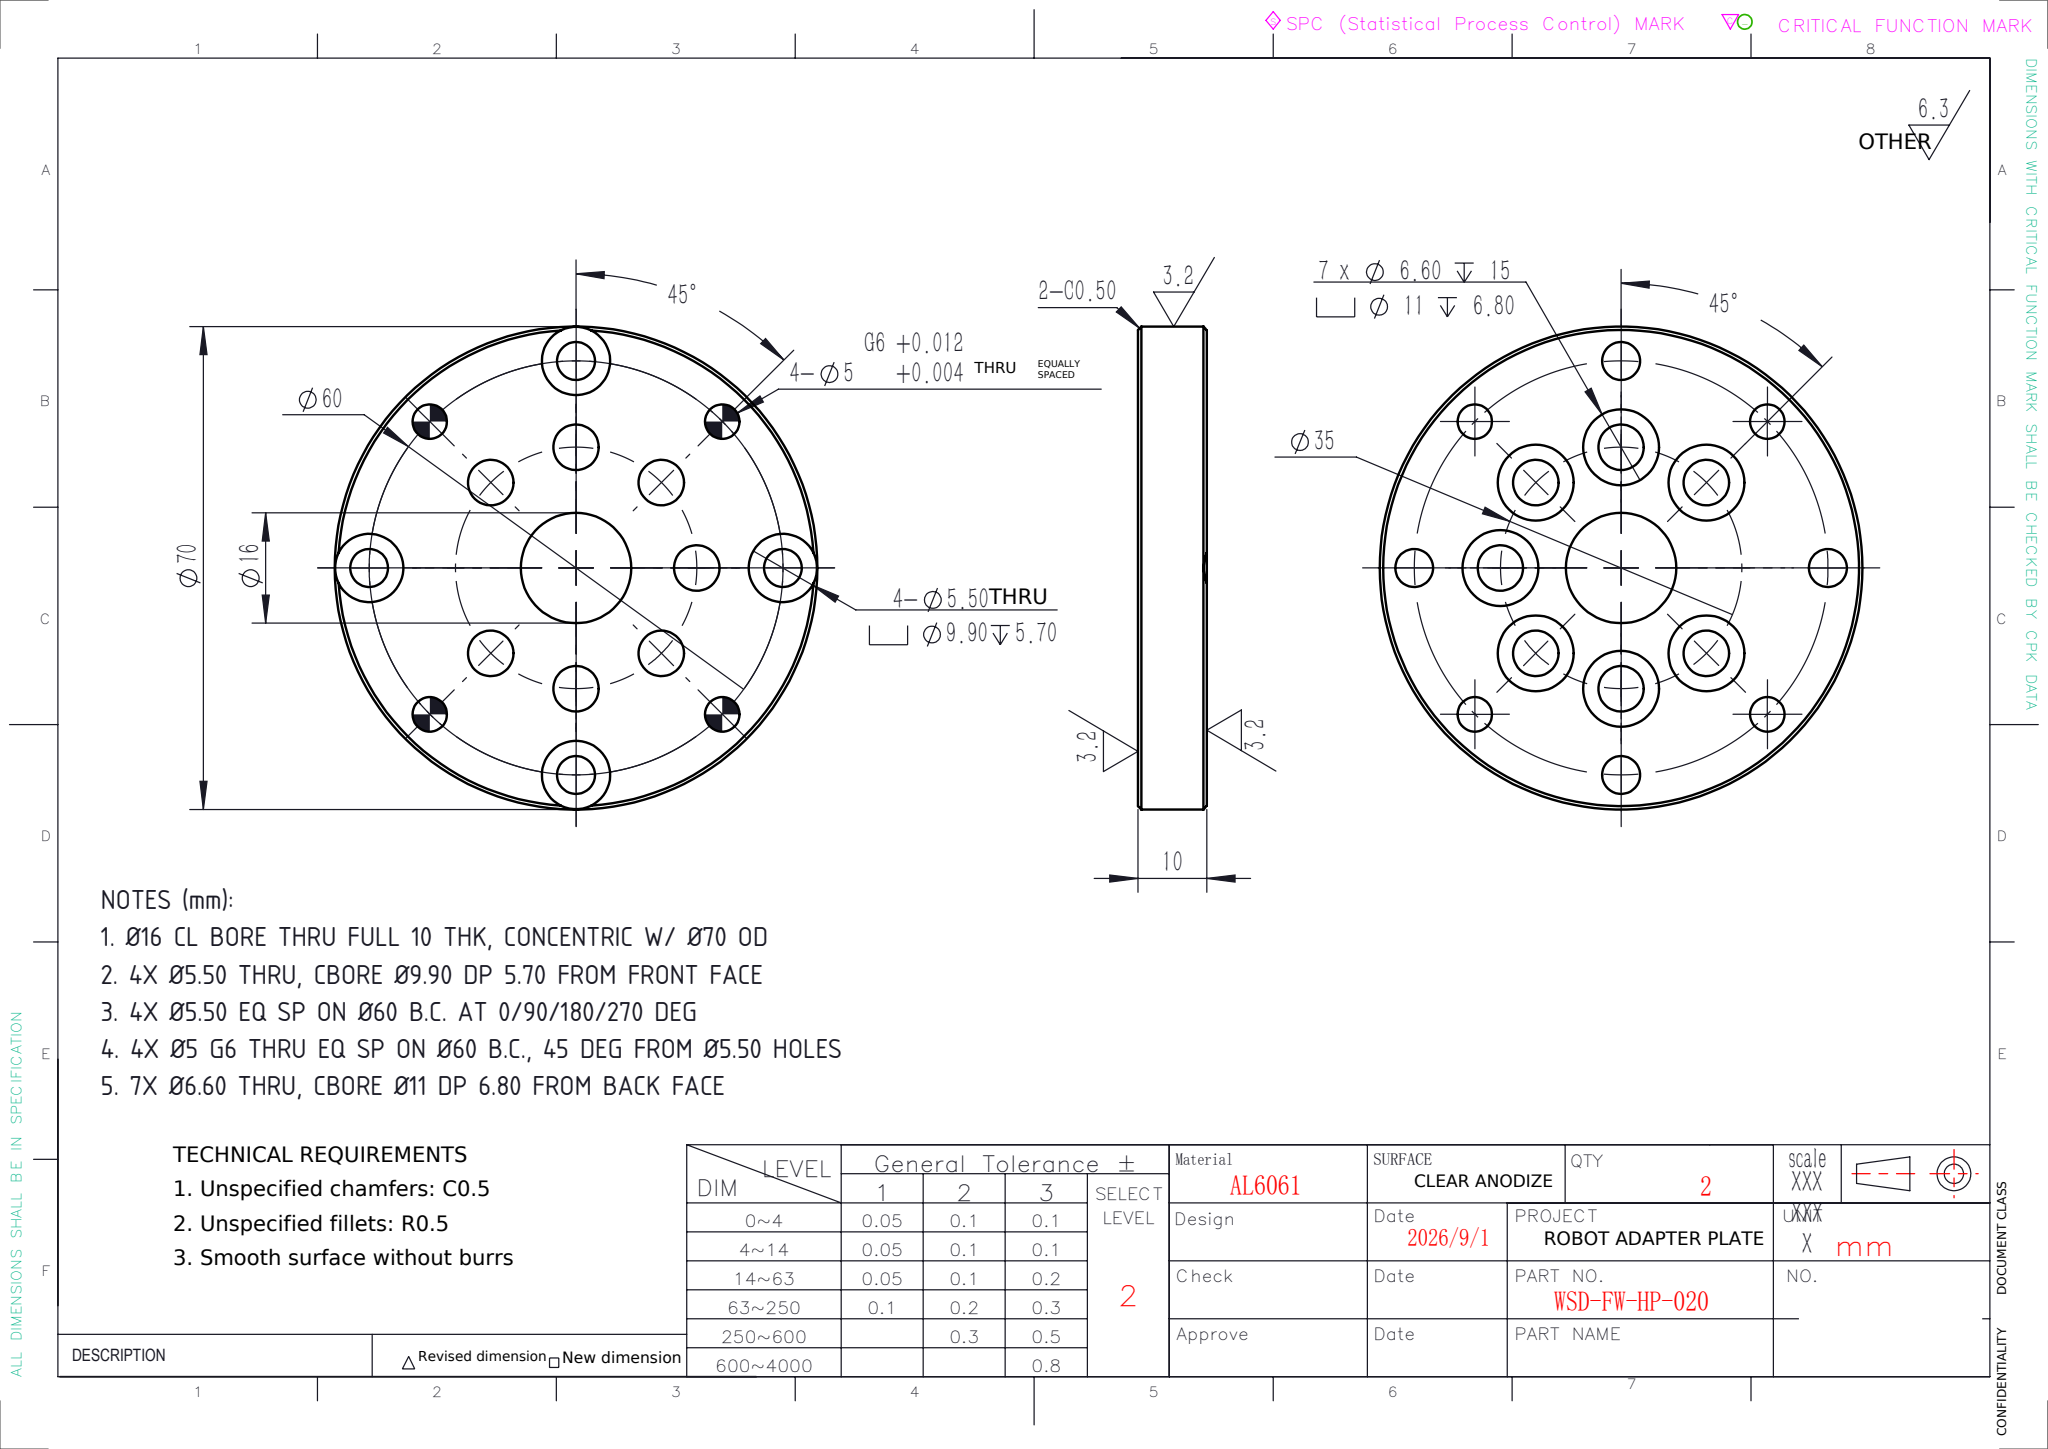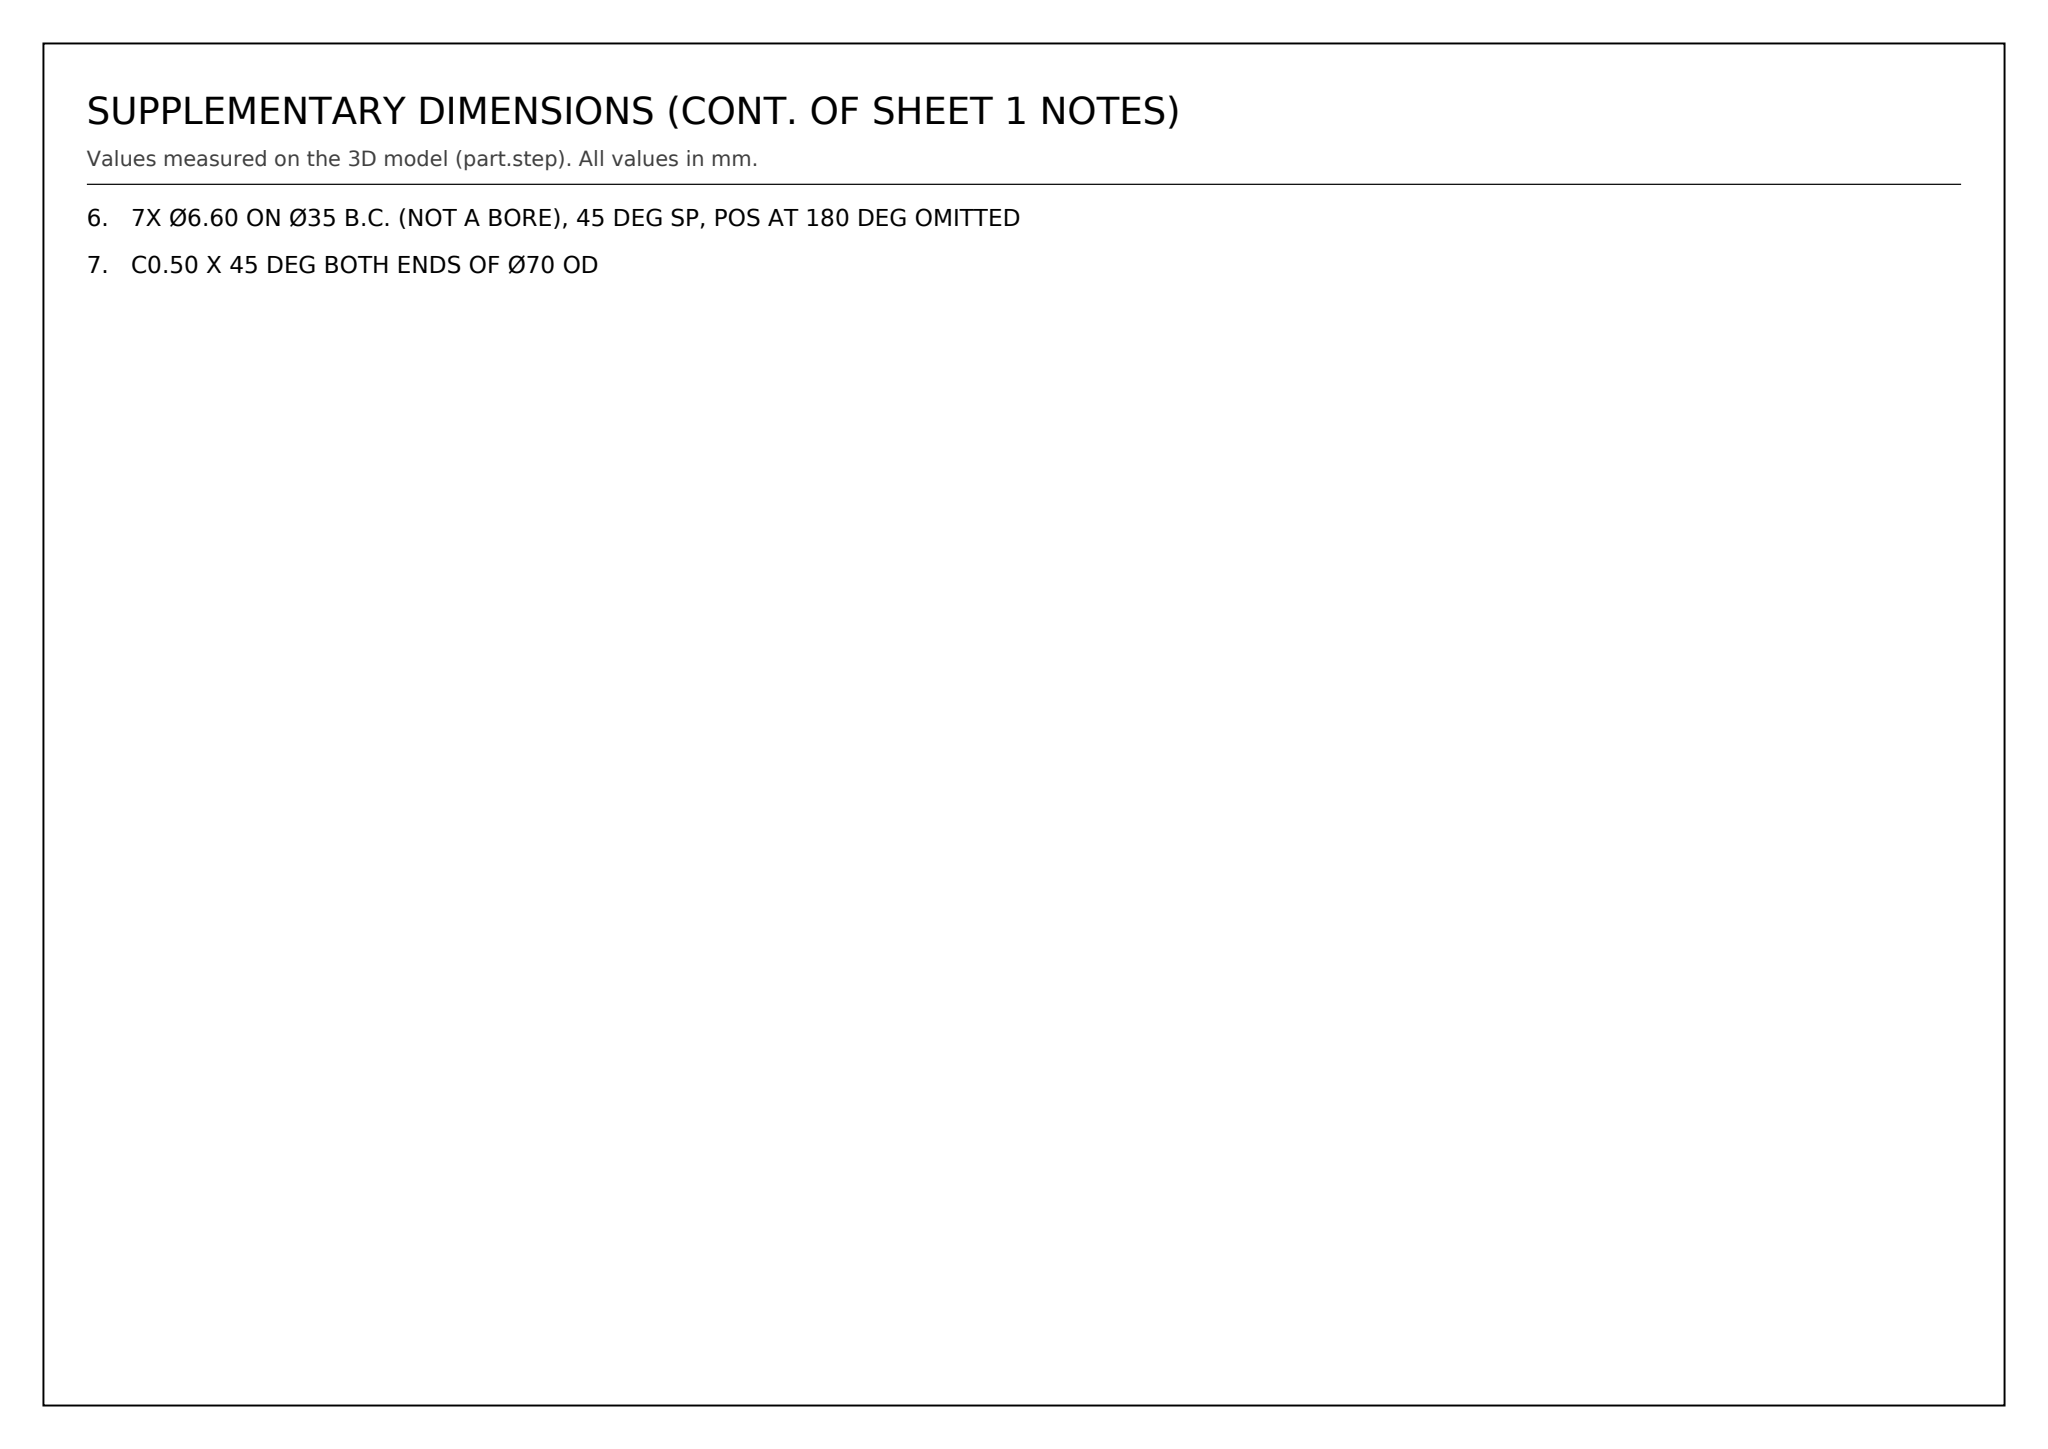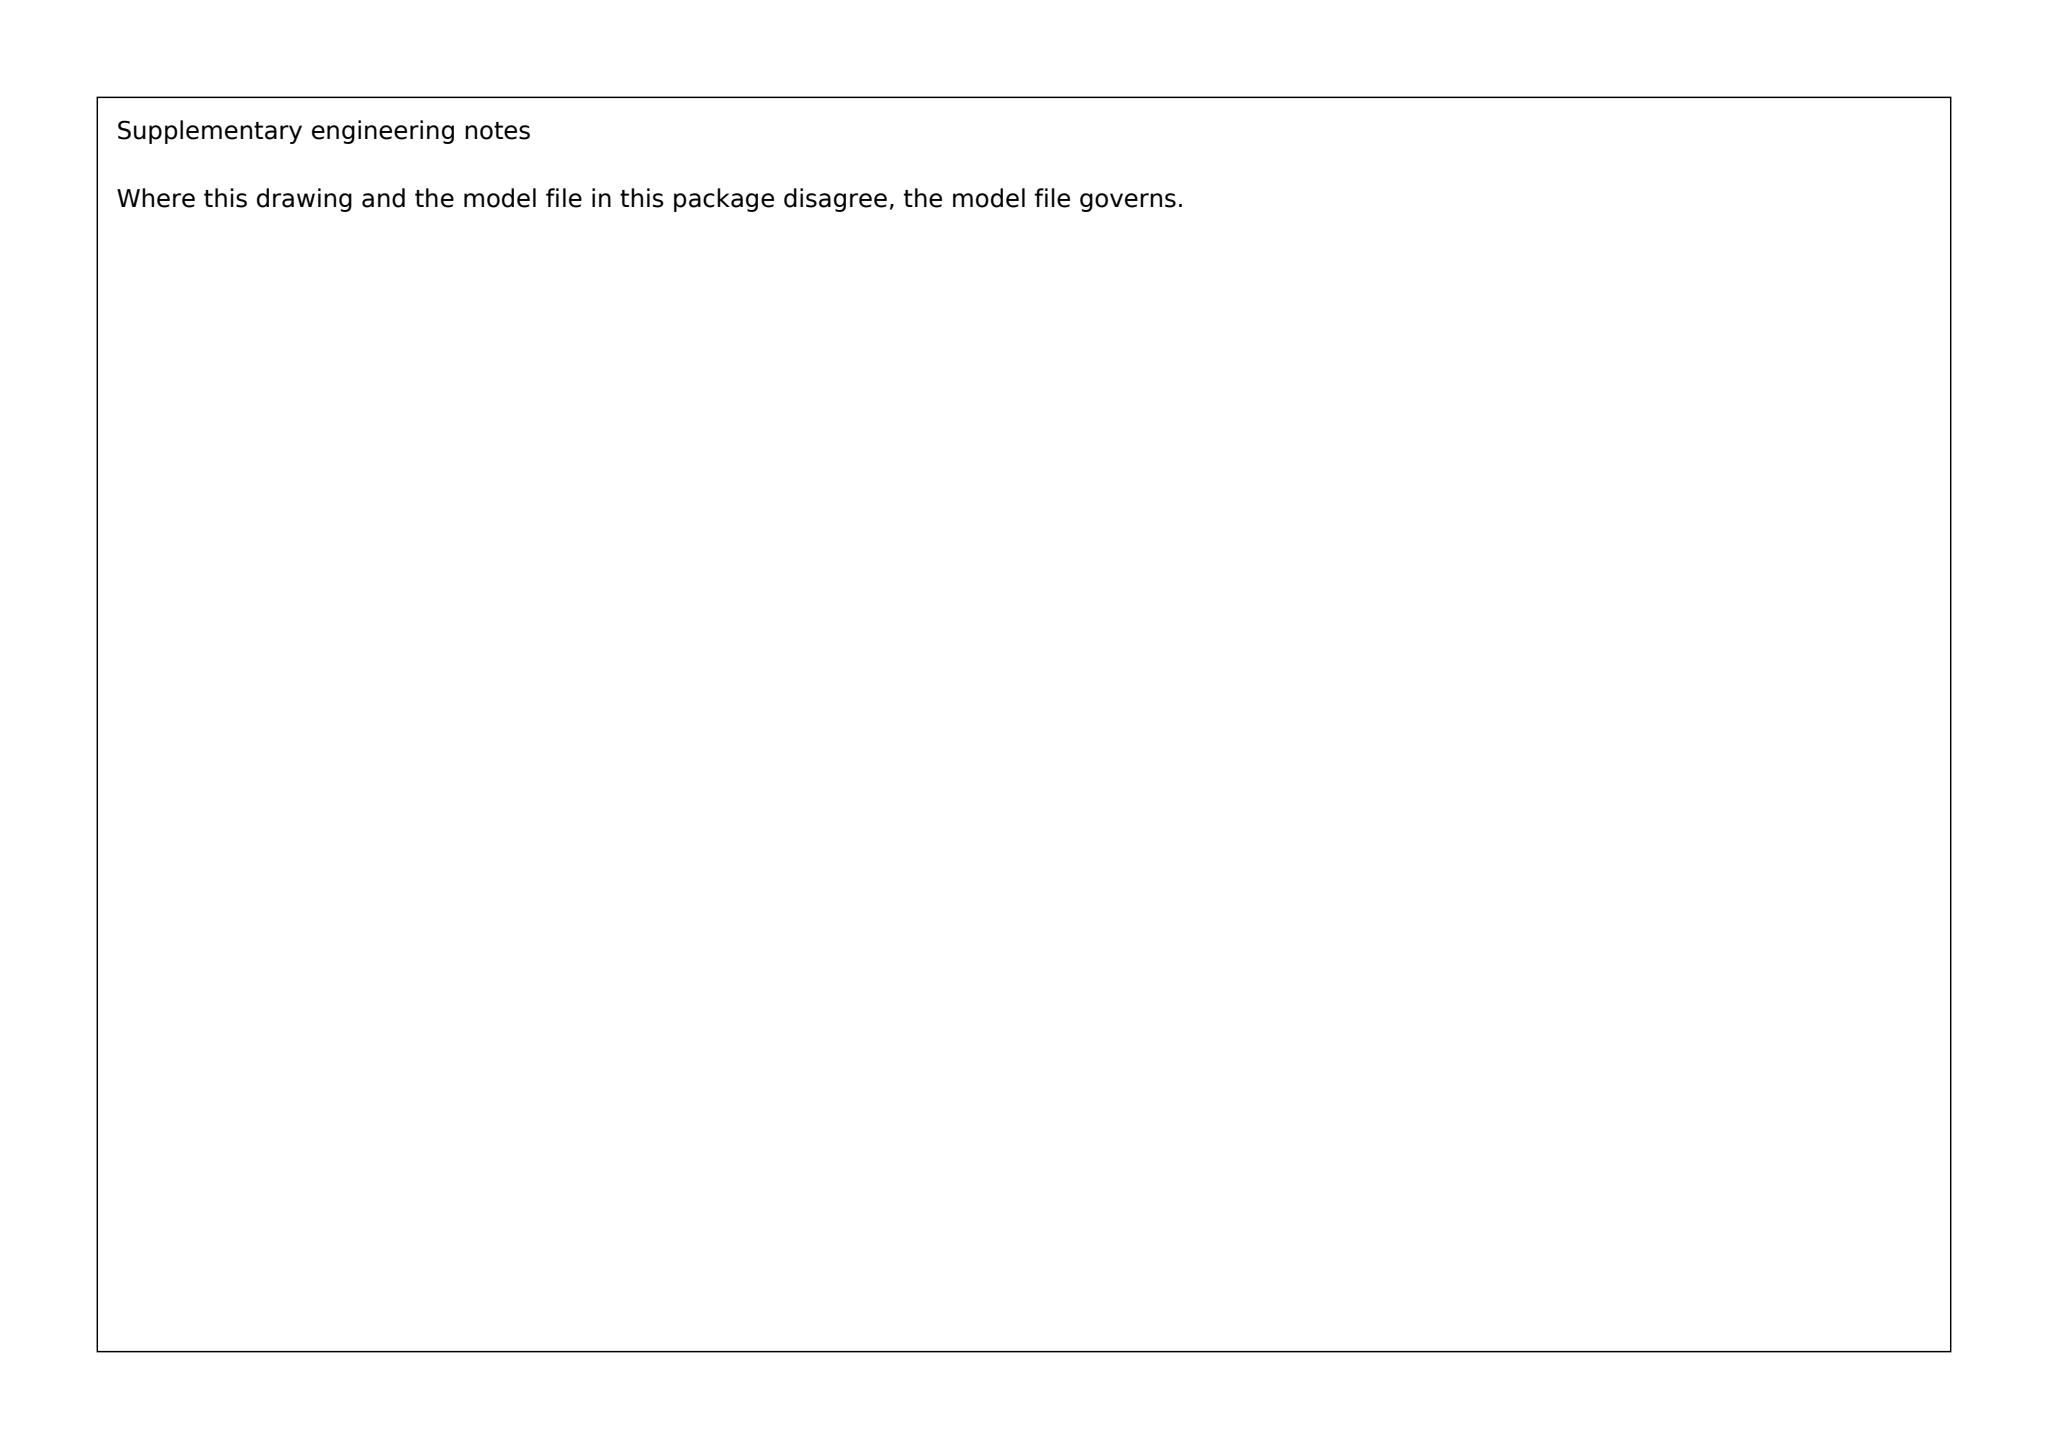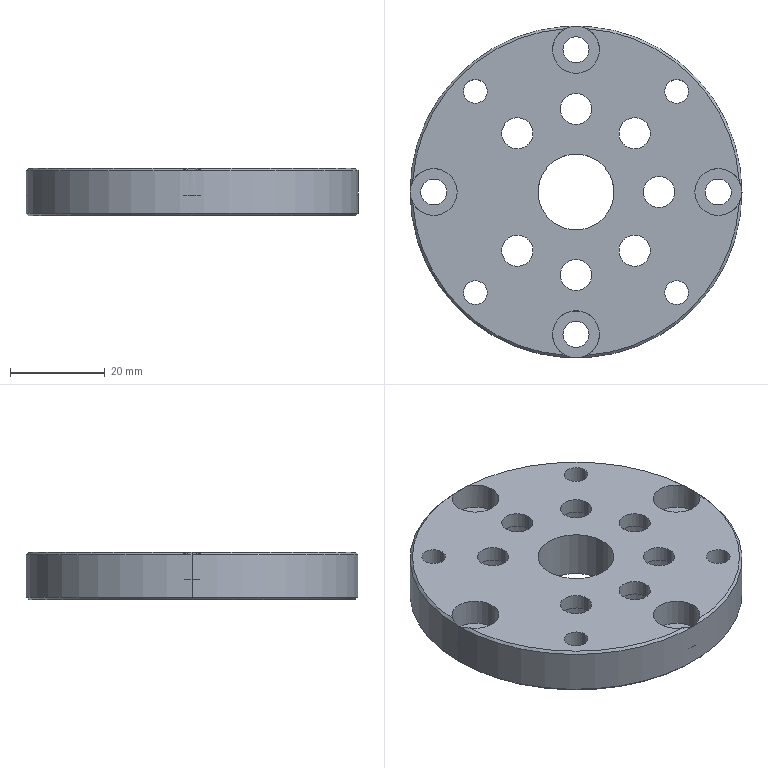Part | SolidWorks | mm | 1 solid | 73 faces | box 70 x 70 x 10 mm | volume 28181 mm3 | cylinder 56 | plane 13 | cone 4 | commonest cylinder face diameters 11 x14 6.6 x14 5 x8 9.9 x8 5.5 x8 16 x2 70 x2
Drawing notes:
Ø16 CL BORE THRU FULL 10 THK, CONCENTRIC W/ Ø70 OD | from the solid: Ø16 cyl at (35,35), length 10 = full thickness
4X Ø5.50 THRU, CBORE Ø9.90 DP 5.70 FROM FRONT FACE | from the solid: Ø5.5 len 4.3 + Ø9.9 len 5.7 = 10 thru; plane z=4.3
4X Ø5.50 EQ SP ON Ø60 B.C. AT 0/90/180/270 DEG | from the solid: Ø5.5 holes at (5,35),(35,5),(35,65),(65,35); center (35,35) -> R30
4X Ø5 G6 THRU EQ SP ON Ø60 B.C., 45 DEG FROM Ø5.50 HOLES | from the solid: Ø5 holes at (13.79,13.79) etc -> R30.0 at 45/135/225/315 deg
7X Ø6.60 THRU, CBORE Ø11 DP 6.80 FROM BACK FACE | from the solid: Ø6.6 len 3.2 + Ø11 len 6.8 = 10 thru; CBORE from z=0 face
7X Ø6.60 ON Ø35 B.C. (NOT A BORE), 45 DEG SP, POS AT 180 DEG OMITTED | from the solid: Ø6.6 at (52.5,35),(47.37,47.37),(35,52.5),(22.63,47.37),(22.63,22.63),(35,17.5),(47.37,22.63); R17.5; no Ø35 cyl
C0.50 X 45 DEG BOTH ENDS OF Ø70 OD | from the solid: cones 90 deg incl, ref dia 69 and 70, 2 ea